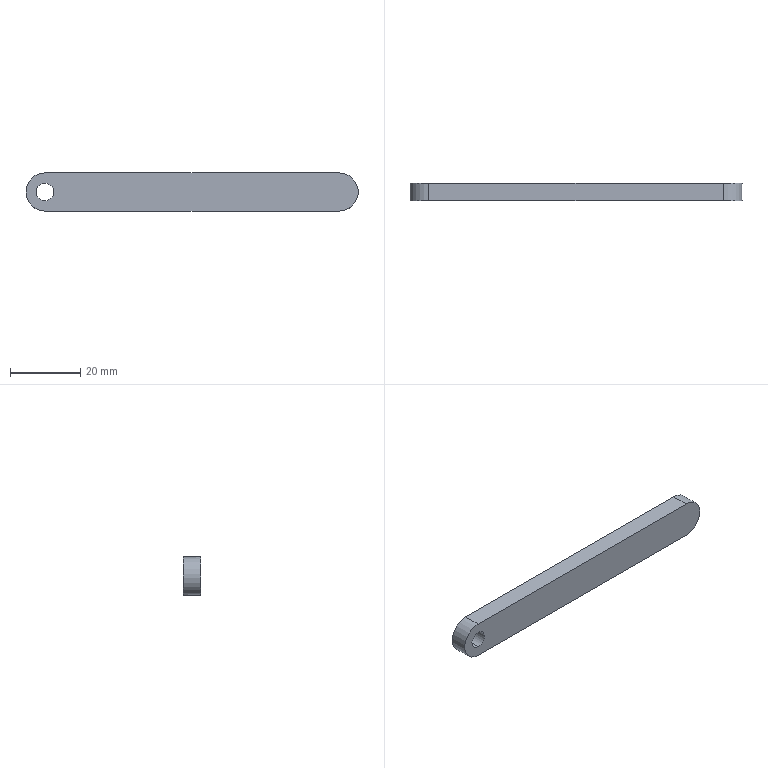Component | SolidWorks | RehabilitationChair-18-14-4 | 1 solid | 8 faces | box 94.86 x 5.04 x 10.89 mm | volume 4930 mm3 | cylinder 4 | plane 4 | commonest cylinder face diameters 5.024 x2 10.87 x2
STEP:
#1=CARTESIAN_POINT('',(16.416,6.261,11.67));
#2=VERTEX_POINT('',#1);
#3=CARTESIAN_POINT('',(16.416,6.262,11.868));
#4=VERTEX_POINT('',#3);
#5=CARTESIAN_POINT('',(16.416,6.261,11.769));
#6=DIRECTION('',(0.,1.,-0.003798));
#7=DIRECTION('',(0.,0.003798,1.));
#8=AXIS2_PLACEMENT_3D('',#5,#6,#7);
#9=CIRCLE('',#8,0.0989);
#10=EDGE_CURVE('',#2,#4,#9,.T.);
#11=ORIENTED_EDGE('',*,*,#10,.F.);
#12=CARTESIAN_POINT('',(16.416,6.458,11.67));
#13=VERTEX_POINT('',#12);
#14=CARTESIAN_POINT('',(16.416,5.053,11.675));
#15=DIRECTION('',(0.,1.,-0.003798));
#16=VECTOR('',#15,39.37);
#17=LINE('',#14,#16);
#18=EDGE_CURVE('',#2,#13,#17,.T.);
#19=ORIENTED_EDGE('',*,*,#18,.T.);
#20=CARTESIAN_POINT('',(16.416,6.459,11.867));
#21=VERTEX_POINT('',#20);
#22=CARTESIAN_POINT('',(16.416,6.458,11.768));
#23=DIRECTION('',(0.,1.,-0.003798));
#24=DIRECTION('',(0.,0.003798,1.));
#25=AXIS2_PLACEMENT_3D('',#22,#23,#24);
#26=CIRCLE('',#25,0.0989);
#27=EDGE_CURVE('',#13,#21,#26,.T.);
#28=ORIENTED_EDGE('',*,*,#27,.T.);
#29=CARTESIAN_POINT('',(16.416,5.054,11.873));
#30=DIRECTION('',(0.,1.,-0.003798));
#31=VECTOR('',#30,39.37);
#32=LINE('',#29,#31);
#33=EDGE_CURVE('',#4,#21,#32,.T.);
#34=ORIENTED_EDGE('',*,*,#33,.F.);
#35=EDGE_LOOP('',(#11,#19,#28,#34));
#36=FACE_OUTER_BOUND('',#35,.T.);
#37=CARTESIAN_POINT('',(16.416,5.054,11.774));
#38=DIRECTION('',(0.,1.,-0.003798));
#39=DIRECTION('',(0.,0.003798,1.));
#40=AXIS2_PLACEMENT_3D('',#37,#38,#39);
#41=CYLINDRICAL_SURFACE('',#40,0.0989);
#42=ADVANCED_FACE('',(#36),#41,.F.);
#43=ORIENTED_EDGE('',*,*,#18,.F.);
#44=CARTESIAN_POINT('',(16.416,6.261,11.769));
#45=DIRECTION('',(0.,1.,-0.003798));
#46=DIRECTION('',(0.,0.003798,1.));
#47=AXIS2_PLACEMENT_3D('',#44,#45,#46);
#48=CIRCLE('',#47,0.0989);
#49=EDGE_CURVE('',#4,#2,#48,.T.);
#50=ORIENTED_EDGE('',*,*,#49,.F.);
#51=ORIENTED_EDGE('',*,*,#33,.T.);
#52=CARTESIAN_POINT('',(16.416,6.458,11.768));
#53=DIRECTION('',(0.,1.,-0.003798));
#54=DIRECTION('',(0.,0.003798,1.));
#55=AXIS2_PLACEMENT_3D('',#52,#53,#54);
#56=CIRCLE('',#55,0.0989);
#57=EDGE_CURVE('',#21,#13,#56,.T.);
#58=ORIENTED_EDGE('',*,*,#57,.T.);
#59=EDGE_LOOP('',(#43,#50,#51,#58));
#60=FACE_OUTER_BOUND('',#59,.T.);
#61=CARTESIAN_POINT('',(16.416,5.054,11.774));
#62=DIRECTION('',(0.,1.,-0.003798));
#63=DIRECTION('',(0.,0.003798,1.));
#64=AXIS2_PLACEMENT_3D('',#61,#62,#63);
#65=CYLINDRICAL_SURFACE('',#64,0.0989);
#66=ADVANCED_FACE('',(#60),#65,.F.);
#67=ORIENTED_EDGE('',*,*,#57,.F.);
#68=ORIENTED_EDGE('',*,*,#27,.F.);
#69=EDGE_LOOP('',(#67,#68));
#70=FACE_BOUND('',#69,.T.);
#71=CARTESIAN_POINT('',(16.416,6.457,11.554));
#72=VERTEX_POINT('',#71);
#73=CARTESIAN_POINT('',(16.416,6.459,11.982));
#74=VERTEX_POINT('',#73);
#75=CARTESIAN_POINT('',(16.416,6.458,11.768));
#76=DIRECTION('',(0.,1.,-0.003798));
#77=DIRECTION('',(0.,0.003798,1.));
#78=AXIS2_PLACEMENT_3D('',#75,#76,#77);
#79=CIRCLE('',#78,0.214);
#80=EDGE_CURVE('',#72,#74,#79,.T.);
#81=ORIENTED_EDGE('',*,*,#80,.T.);
#82=CARTESIAN_POINT('',(19.723,6.459,11.982));
#83=VERTEX_POINT('',#82);
#84=CARTESIAN_POINT('',(16.416,6.459,11.982));
#85=DIRECTION('',(1.,-0.,0.));
#86=VECTOR('',#85,39.37);
#87=LINE('',#84,#86);
#88=EDGE_CURVE('',#74,#83,#87,.T.);
#89=ORIENTED_EDGE('',*,*,#88,.T.);
#90=CARTESIAN_POINT('',(19.723,6.457,11.554));
#91=VERTEX_POINT('',#90);
#92=CARTESIAN_POINT('',(19.723,6.458,11.768));
#93=DIRECTION('',(0.,1.,-0.003798));
#94=DIRECTION('',(0.,0.003798,1.));
#95=AXIS2_PLACEMENT_3D('',#92,#93,#94);
#96=CIRCLE('',#95,0.214);
#97=EDGE_CURVE('',#83,#91,#96,.T.);
#98=ORIENTED_EDGE('',*,*,#97,.T.);
#99=CARTESIAN_POINT('',(16.416,6.457,11.554));
#100=DIRECTION('',(-1.,0.,-0.));
#101=VECTOR('',#100,39.37);
#102=LINE('',#99,#101);
#103=EDGE_CURVE('',#91,#72,#102,.T.);
#104=ORIENTED_EDGE('',*,*,#103,.T.);
#105=EDGE_LOOP('',(#81,#89,#98,#104));
#106=FACE_OUTER_BOUND('',#105,.T.);
#107=CARTESIAN_POINT('',(16.416,6.458,11.768));
#108=DIRECTION('',(0.,1.,-0.003798));
#109=DIRECTION('',(-0.,0.003798,1.));
#110=AXIS2_PLACEMENT_3D('',#107,#108,#109);
#111=PLANE('',#110);
#112=ADVANCED_FACE('',(#70,#106),#111,.T.);
#113=ORIENTED_EDGE('',*,*,#49,.T.);
#114=ORIENTED_EDGE('',*,*,#10,.T.);
#115=EDGE_LOOP('',(#113,#114));
#116=FACE_BOUND('',#115,.T.);
#117=CARTESIAN_POINT('',(16.416,6.261,11.555));
#118=VERTEX_POINT('',#117);
#119=CARTESIAN_POINT('',(16.416,6.262,11.983));
#120=VERTEX_POINT('',#119);
#121=CARTESIAN_POINT('',(16.416,6.261,11.769));
#122=DIRECTION('',(0.,1.,-0.003798));
#123=DIRECTION('',(0.,0.003798,1.));
#124=AXIS2_PLACEMENT_3D('',#121,#122,#123);
#125=CIRCLE('',#124,0.214);
#126=EDGE_CURVE('',#118,#120,#125,.T.);
#127=ORIENTED_EDGE('',*,*,#126,.F.);
#128=CARTESIAN_POINT('',(19.723,6.261,11.555));
#129=VERTEX_POINT('',#128);
#130=CARTESIAN_POINT('',(16.416,6.261,11.555));
#131=DIRECTION('',(-1.,0.,-0.));
#132=VECTOR('',#131,39.37);
#133=LINE('',#130,#132);
#134=EDGE_CURVE('',#129,#118,#133,.T.);
#135=ORIENTED_EDGE('',*,*,#134,.F.);
#136=CARTESIAN_POINT('',(19.723,6.262,11.983));
#137=VERTEX_POINT('',#136);
#138=CARTESIAN_POINT('',(19.723,6.261,11.769));
#139=DIRECTION('',(0.,1.,-0.003798));
#140=DIRECTION('',(0.,0.003798,1.));
#141=AXIS2_PLACEMENT_3D('',#138,#139,#140);
#142=CIRCLE('',#141,0.214);
#143=EDGE_CURVE('',#137,#129,#142,.T.);
#144=ORIENTED_EDGE('',*,*,#143,.F.);
#145=CARTESIAN_POINT('',(16.416,6.262,11.983));
#146=DIRECTION('',(1.,-0.,0.));
#147=VECTOR('',#146,39.37);
#148=LINE('',#145,#147);
#149=EDGE_CURVE('',#120,#137,#148,.T.);
#150=ORIENTED_EDGE('',*,*,#149,.F.);
#151=EDGE_LOOP('',(#127,#135,#144,#150));
#152=FACE_OUTER_BOUND('',#151,.T.);
#153=CARTESIAN_POINT('',(16.416,6.261,11.769));
#154=DIRECTION('',(0.,1.,-0.003798));
#155=DIRECTION('',(-0.,0.003798,1.));
#156=AXIS2_PLACEMENT_3D('',#153,#154,#155);
#157=PLANE('',#156);
#158=ADVANCED_FACE('',(#116,#152),#157,.F.);
#159=ORIENTED_EDGE('',*,*,#126,.T.);
#160=CARTESIAN_POINT('',(16.416,6.459,11.982));
#161=DIRECTION('',(-0.,-1.,0.003798));
#162=VECTOR('',#161,39.37);
#163=LINE('',#160,#162);
#164=EDGE_CURVE('',#74,#120,#163,.T.);
#165=ORIENTED_EDGE('',*,*,#164,.F.);
#166=ORIENTED_EDGE('',*,*,#80,.F.);
#167=CARTESIAN_POINT('',(16.416,6.457,11.554));
#168=DIRECTION('',(-0.,-1.,0.003798));
#169=VECTOR('',#168,39.37);
#170=LINE('',#167,#169);
#171=EDGE_CURVE('',#72,#118,#170,.T.);
#172=ORIENTED_EDGE('',*,*,#171,.T.);
#173=EDGE_LOOP('',(#159,#165,#166,#172));
#174=FACE_OUTER_BOUND('',#173,.T.);
#175=CARTESIAN_POINT('',(16.416,6.458,11.768));
#176=DIRECTION('',(-0.,-1.,0.003798));
#177=DIRECTION('',(0.,-0.003798,-1.));
#178=AXIS2_PLACEMENT_3D('',#175,#176,#177);
#179=CYLINDRICAL_SURFACE('',#178,0.214);
#180=ADVANCED_FACE('',(#174),#179,.T.);
#181=ORIENTED_EDGE('',*,*,#134,.T.);
#182=ORIENTED_EDGE('',*,*,#171,.F.);
#183=ORIENTED_EDGE('',*,*,#103,.F.);
#184=CARTESIAN_POINT('',(19.723,6.457,11.554));
#185=DIRECTION('',(-0.,-1.,0.003798));
#186=VECTOR('',#185,39.37);
#187=LINE('',#184,#186);
#188=EDGE_CURVE('',#91,#129,#187,.T.);
#189=ORIENTED_EDGE('',*,*,#188,.T.);
#190=EDGE_LOOP('',(#181,#182,#183,#189));
#191=FACE_OUTER_BOUND('',#190,.T.);
#192=CARTESIAN_POINT('',(16.416,6.457,11.554));
#193=DIRECTION('',(-0.,0.003798,1.));
#194=DIRECTION('',(-0.,-1.,0.003798));
#195=AXIS2_PLACEMENT_3D('',#192,#193,#194);
#196=PLANE('',#195);
#197=ADVANCED_FACE('',(#191),#196,.F.);
#198=ORIENTED_EDGE('',*,*,#143,.T.);
#199=ORIENTED_EDGE('',*,*,#188,.F.);
#200=ORIENTED_EDGE('',*,*,#97,.F.);
#201=CARTESIAN_POINT('',(19.723,6.459,11.982));
#202=DIRECTION('',(-0.,-1.,0.003798));
#203=VECTOR('',#202,39.37);
#204=LINE('',#201,#203);
#205=EDGE_CURVE('',#83,#137,#204,.T.);
#206=ORIENTED_EDGE('',*,*,#205,.T.);
#207=EDGE_LOOP('',(#198,#199,#200,#206));
#208=FACE_OUTER_BOUND('',#207,.T.);
#209=CARTESIAN_POINT('',(19.723,6.458,11.768));
#210=DIRECTION('',(-0.,-1.,0.003798));
#211=DIRECTION('',(0.,-0.003798,-1.));
#212=AXIS2_PLACEMENT_3D('',#209,#210,#211);
#213=CYLINDRICAL_SURFACE('',#212,0.214);
#214=ADVANCED_FACE('',(#208),#213,.T.);
#215=ORIENTED_EDGE('',*,*,#149,.T.);
#216=ORIENTED_EDGE('',*,*,#205,.F.);
#217=ORIENTED_EDGE('',*,*,#88,.F.);
#218=ORIENTED_EDGE('',*,*,#164,.T.);
#219=EDGE_LOOP('',(#215,#216,#217,#218));
#220=FACE_OUTER_BOUND('',#219,.T.);
#221=CARTESIAN_POINT('',(16.416,6.459,11.982));
#222=DIRECTION('',(0.,-0.003798,-1.));
#223=DIRECTION('',(0.,1.,-0.003798));
#224=AXIS2_PLACEMENT_3D('',#221,#222,#223);
#225=PLANE('',#224);
#226=ADVANCED_FACE('',(#220),#225,.F.);
#227=CLOSED_SHELL('',(#42,#66,#112,#158,#180,#197,#214,#226));
#228=MANIFOLD_SOLID_BREP('',#227);
#229=CARTESIAN_POINT('',(0.,0.,0.));
#230=DIRECTION('',(0.,0.,1.));
#231=DIRECTION('',(1.,0.,0.));
#232=AXIS2_PLACEMENT_3D('',#229,#230,#231);
#233=(LENGTH_UNIT()NAMED_UNIT(*)SI_UNIT($,.METRE.));
#234=LENGTH_MEASURE_WITH_UNIT(LENGTH_MEASURE(0.0254),#233);
#235=DIMENSIONAL_EXPONENTS(1.,0.,0.,0.,0.,0.,0.);
#236=(CONVERSION_BASED_UNIT('',#234)LENGTH_UNIT()NAMED_UNIT(#235));
#237=UNCERTAINTY_MEASURE_WITH_UNIT(LENGTH_MEASURE(0.00001),#236,'','');
#238=(NAMED_UNIT(*)PLANE_ANGLE_UNIT()SI_UNIT($,.RADIAN.));
#239=(NAMED_UNIT(*)SI_UNIT($,.STERADIAN.)SOLID_ANGLE_UNIT());
#240=(GEOMETRIC_REPRESENTATION_CONTEXT(3)GLOBAL_UNCERTAINTY_ASSIGNED_CONTEXT((#237))GLOBAL_UNIT_ASSIGNED_CONTEXT((#236,#238,#239))REPRESENTATION_CONTEXT('',''));
#241=ADVANCED_BREP_SHAPE_REPRESENTATION('',(#228,#232),#240);
#242=COLOUR_RGB('',0.7922,0.8196,0.9333);
#243=FILL_AREA_STYLE_COLOUR('',#242);
#244=FILL_AREA_STYLE('',(#243));
#245=SURFACE_STYLE_FILL_AREA(#244);
#246=SURFACE_SIDE_STYLE('',(#245));
#247=SURFACE_STYLE_USAGE(.BOTH.,#246);
#248=PRESENTATION_STYLE_ASSIGNMENT((#247));
#249=STYLED_ITEM('',(#248),#228);
#250=PRESENTATION_LAYER_ASSIGNMENT('','',(#249));
#251=(LENGTH_UNIT()NAMED_UNIT(*)SI_UNIT($,.METRE.));
#252=LENGTH_MEASURE_WITH_UNIT(LENGTH_MEASURE(0.0254),#251);
#253=DIMENSIONAL_EXPONENTS(1.,0.,0.,0.,0.,0.,0.);
#254=(CONVERSION_BASED_UNIT('',#252)LENGTH_UNIT()NAMED_UNIT(#253));
#255=UNCERTAINTY_MEASURE_WITH_UNIT(LENGTH_MEASURE(0.00001),#254,'','');
#256=(NAMED_UNIT(*)PLANE_ANGLE_UNIT()SI_UNIT($,.RADIAN.));
#257=(NAMED_UNIT(*)SI_UNIT($,.STERADIAN.)SOLID_ANGLE_UNIT());
#258=(GEOMETRIC_REPRESENTATION_CONTEXT(3)GLOBAL_UNCERTAINTY_ASSIGNED_CONTEXT((#255))GLOBAL_UNIT_ASSIGNED_CONTEXT((#254,#256,#257))REPRESENTATION_CONTEXT('',''));
#259=MECHANICAL_DESIGN_GEOMETRIC_PRESENTATION_REPRESENTATION('',(#249),#258);